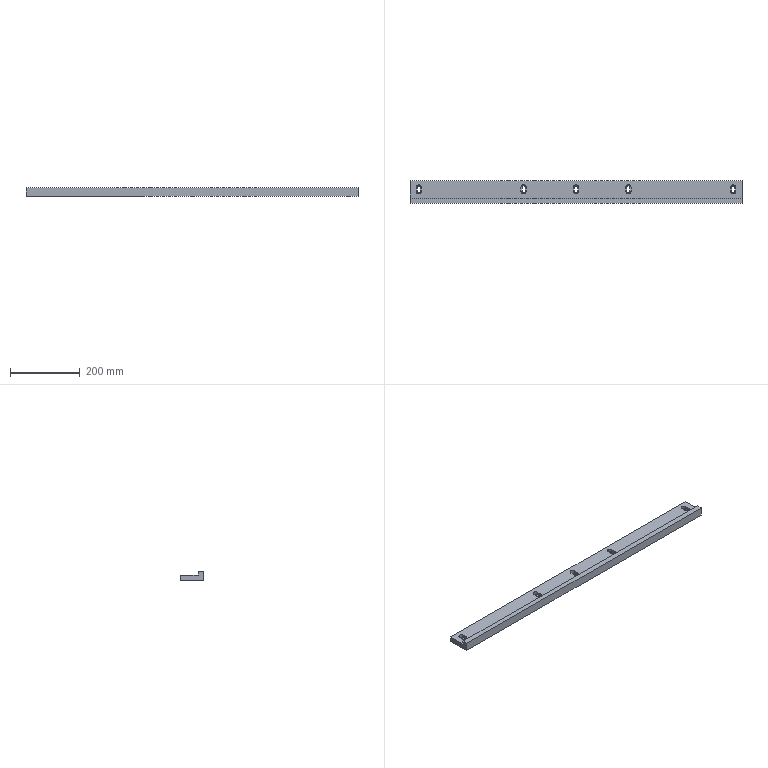Component | SolidWorks | LongFrameSupportA-1 | 1 solid | 63 faces | volume 1048494 mm3 | plane 33 | cylinder 30 | commonest cylinder face diameters 15 x15 9 x15 | material Q235-A